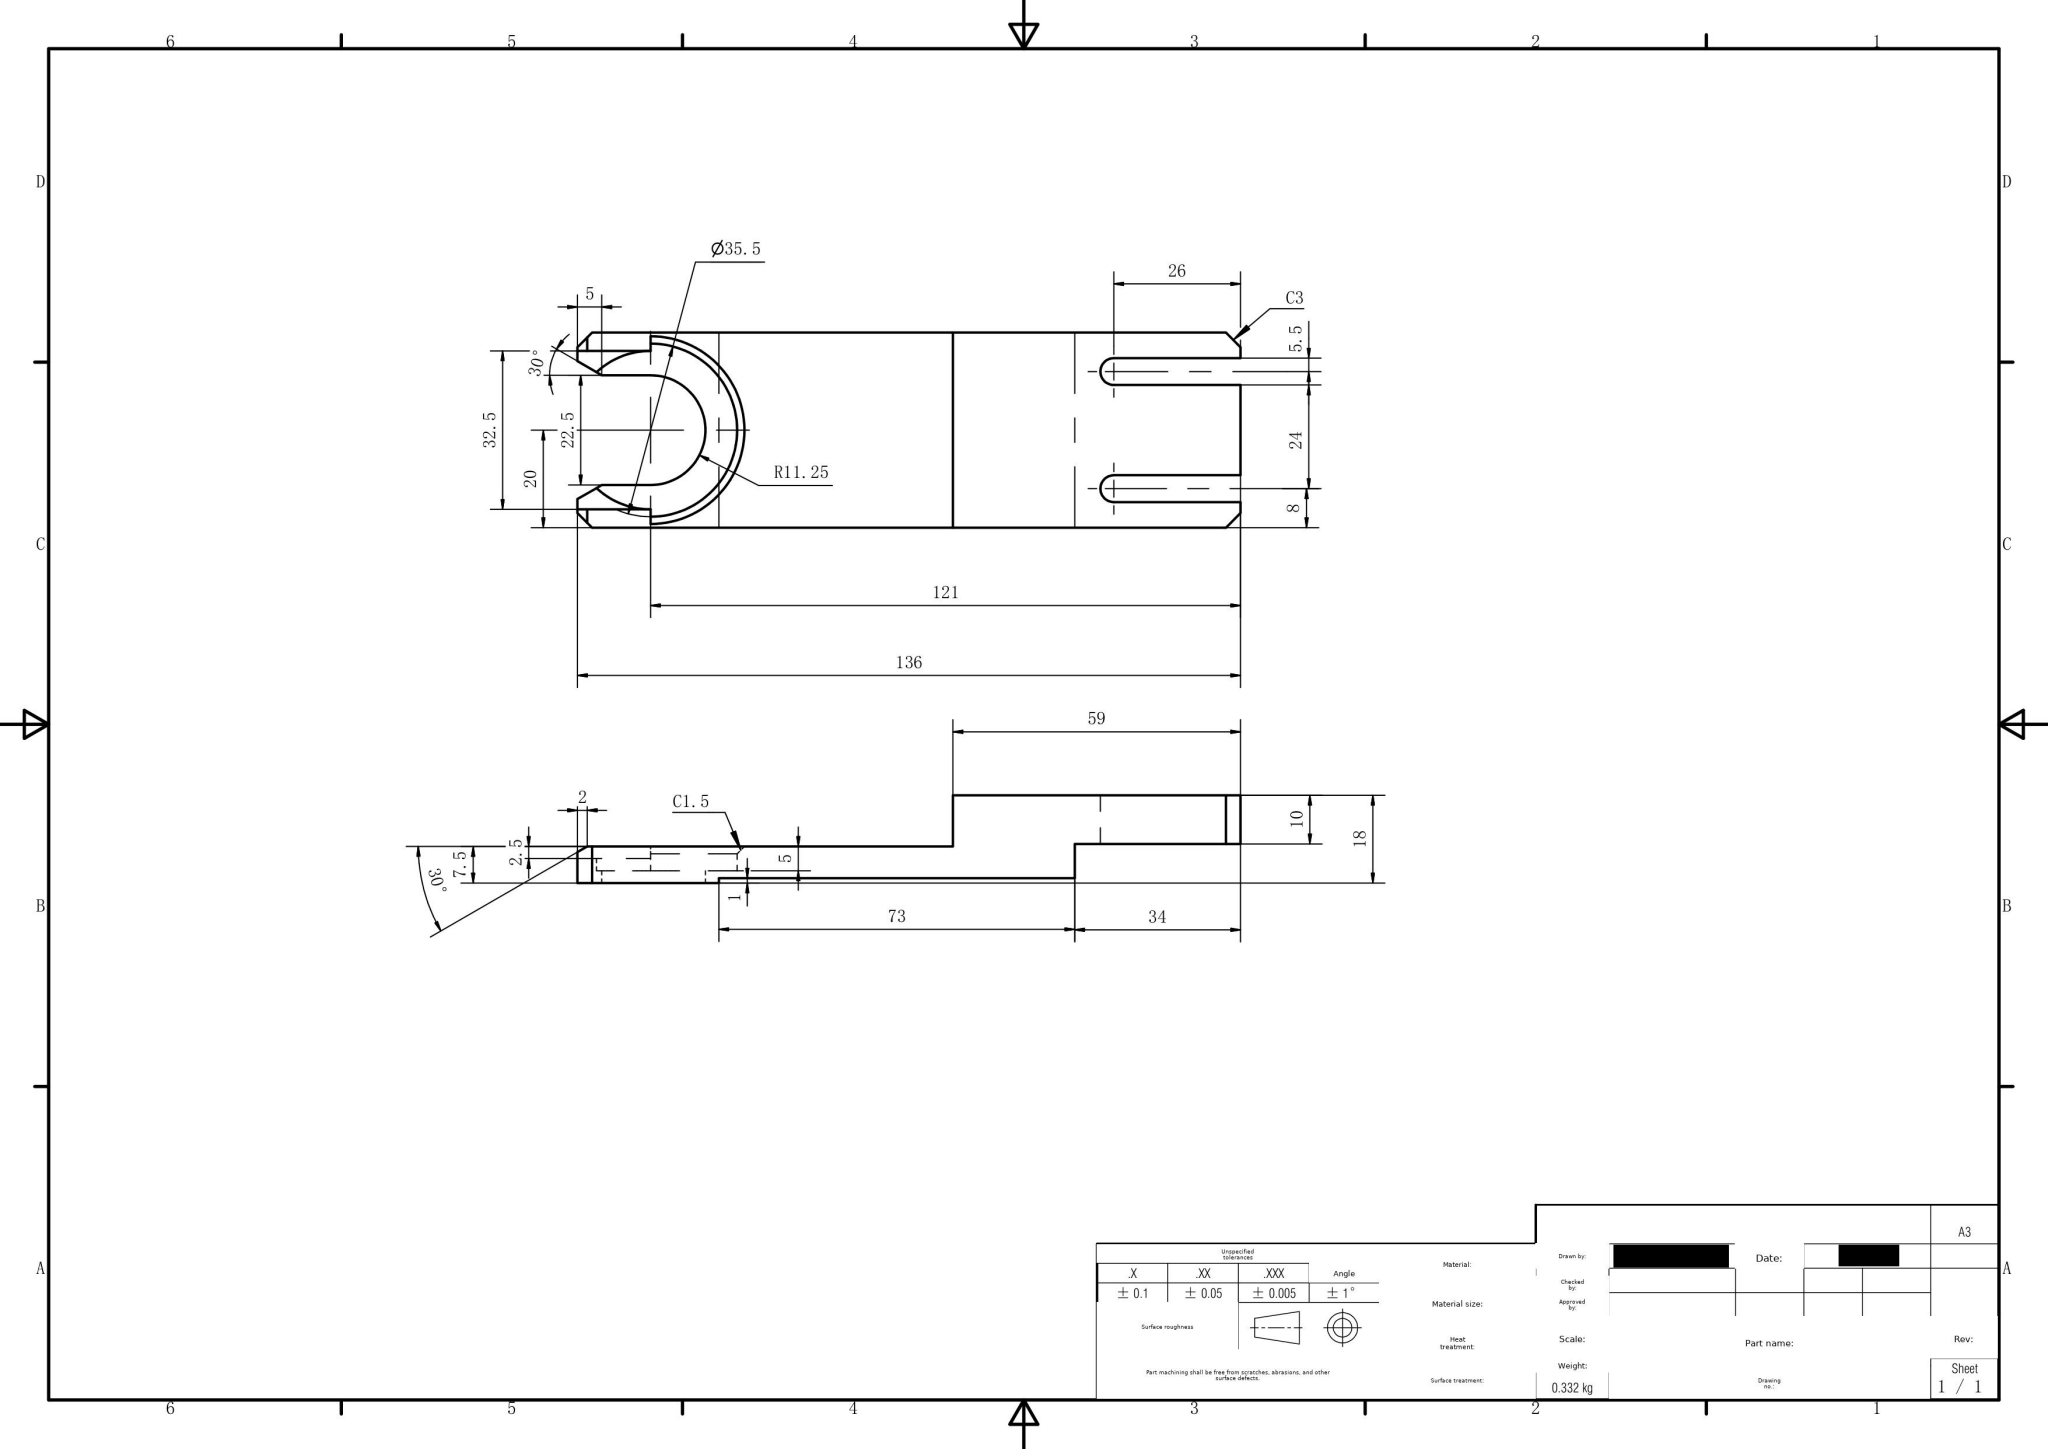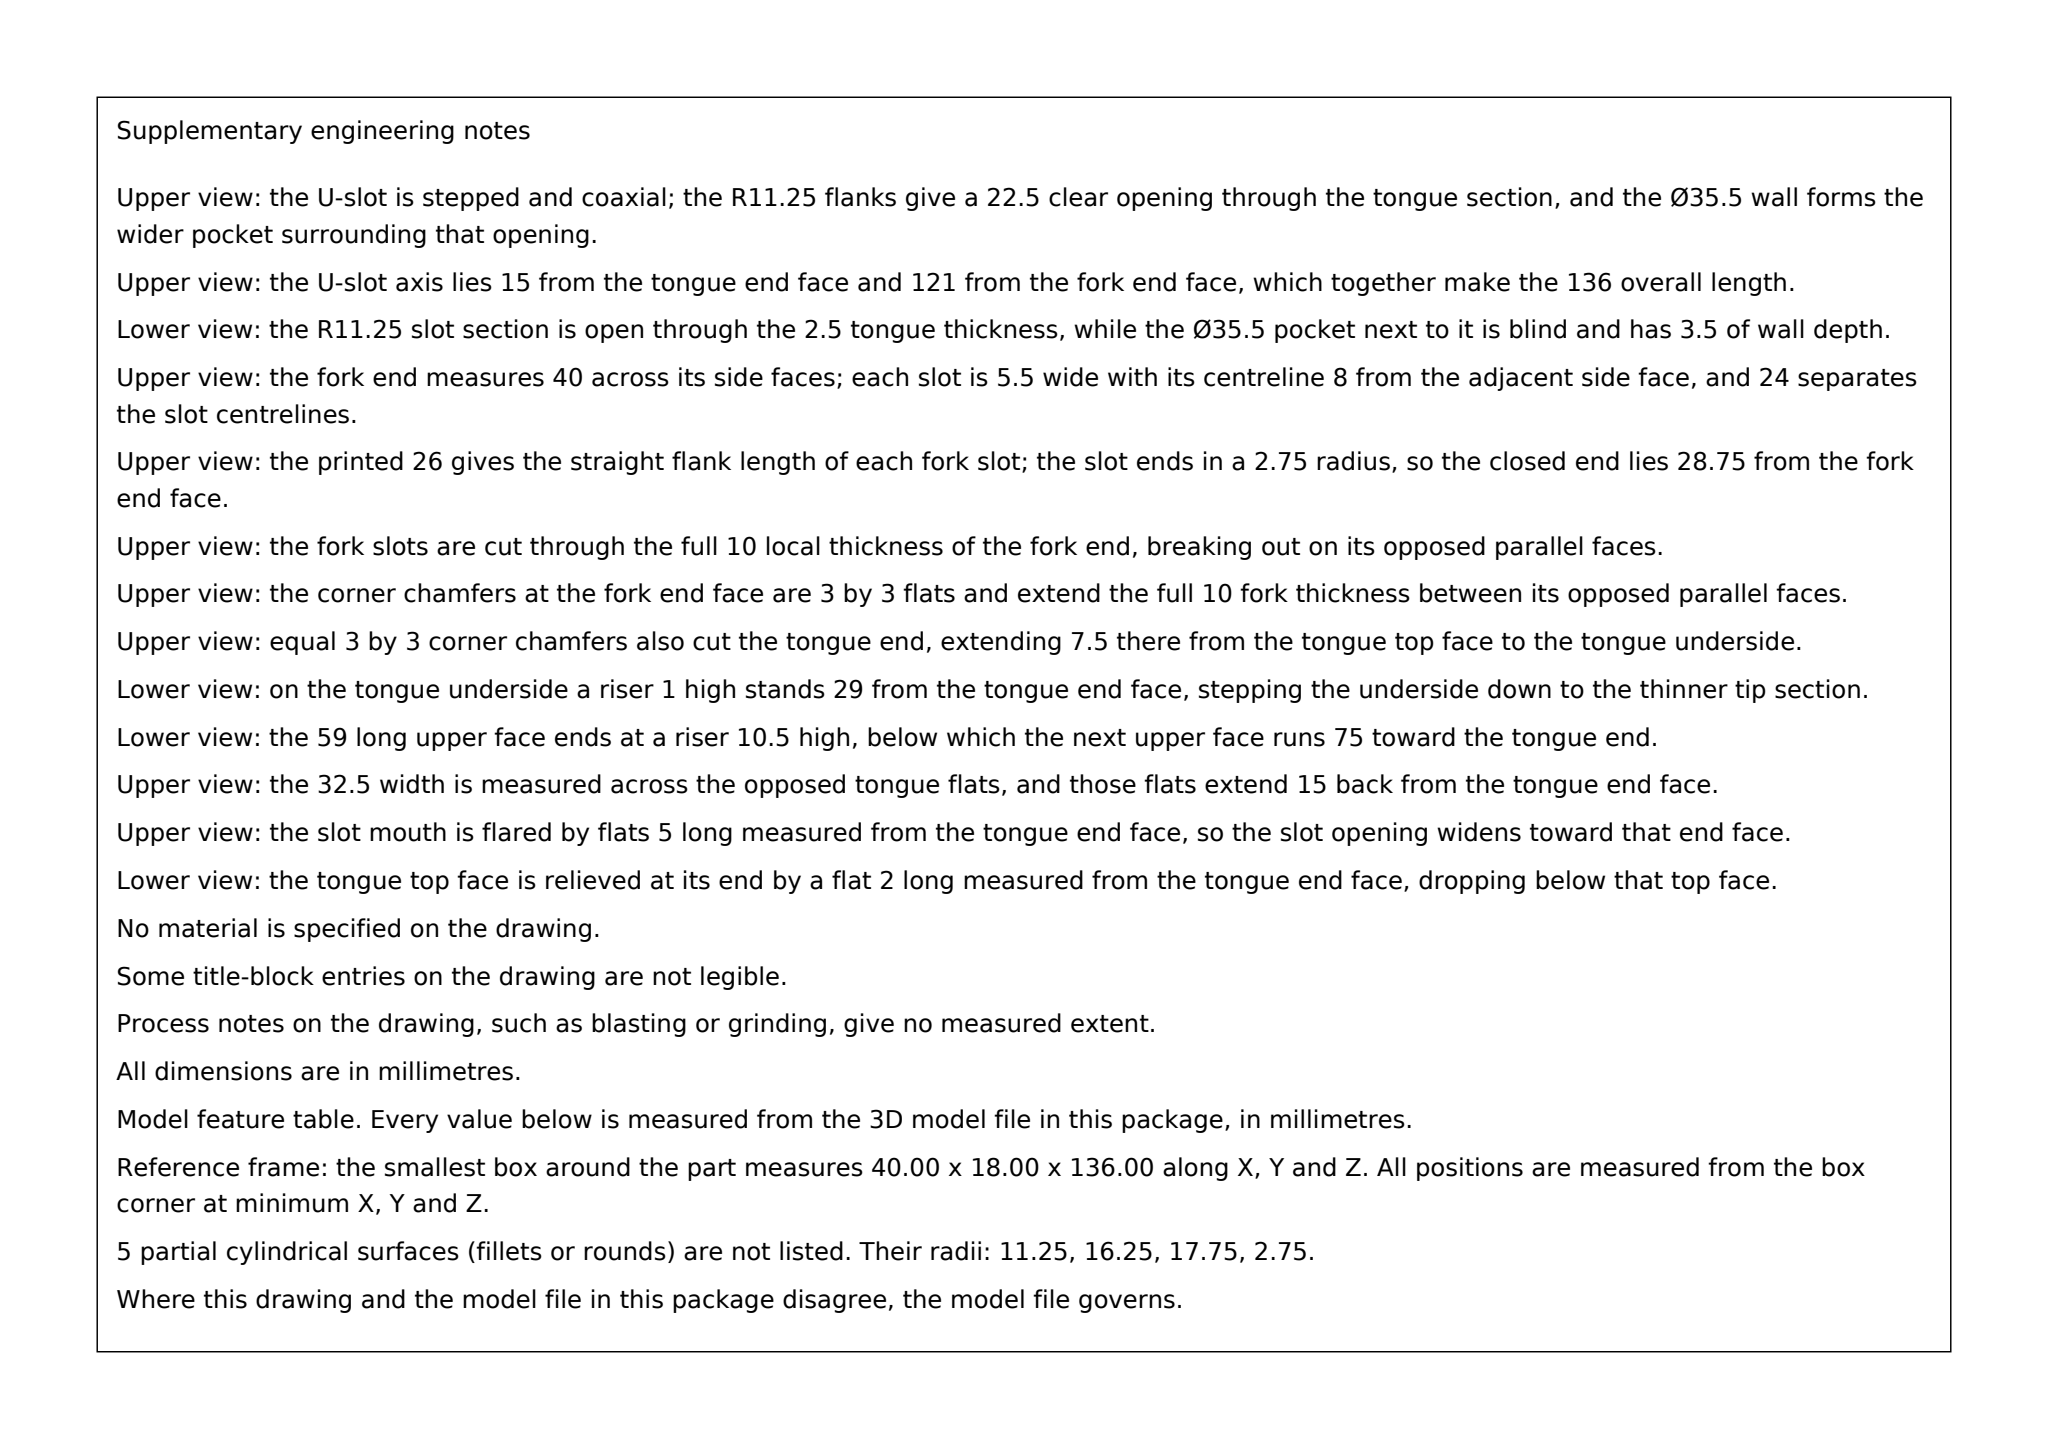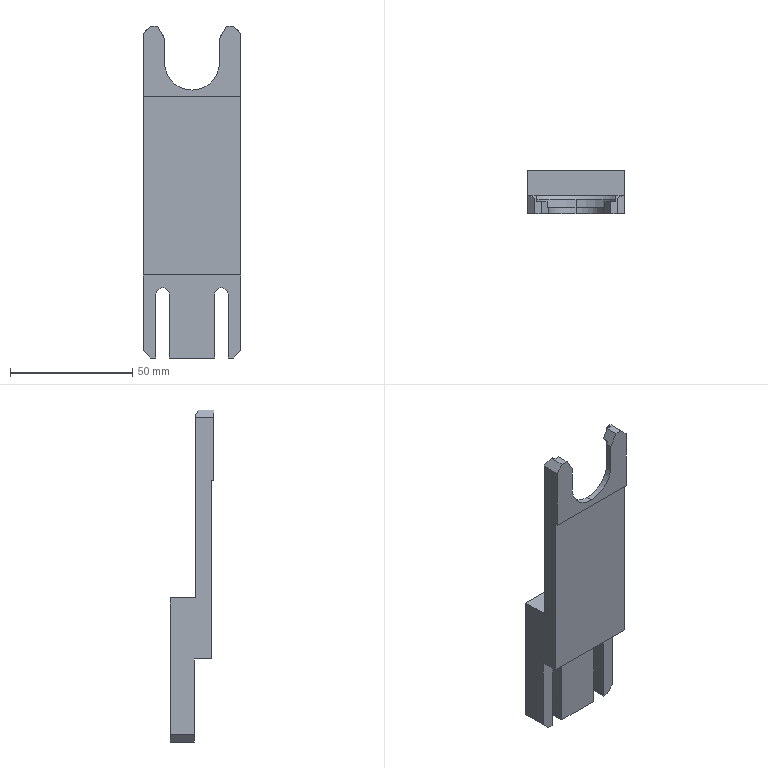Part | SolidWorks | mm | 1 solid | 45 faces | box 40 x 18 x 136 mm | volume 42308 mm3 | plane 36 | cylinder 8 | cone 1 | commonest cylinder face diameters 22.5 x2 35.5 x2 5.5 x2 32.5 x2
Drawing notes:
2X 30° LEAD-IN CHMF AT PRONG TIPS: 5 LG (Z) x 2.9 (X), TIP FACE 3 | from the solid: inclined_planes angle_to_xyz [30,90,60] at bbox_from [5.9,0,131] & [31.2,0,131], size [2.9,5.0,5.0]; z 136 end faces x[3.0,5.9] & [34.1,37.0] = 3 wide
FORK END OUTER CORNERS: 2X C3 (QTY 2, NOT 11) | from the solid: two 45° inclined planes size [3.0,7.5,3.0] at bbox_from [0,0,133] and [37,0,133]